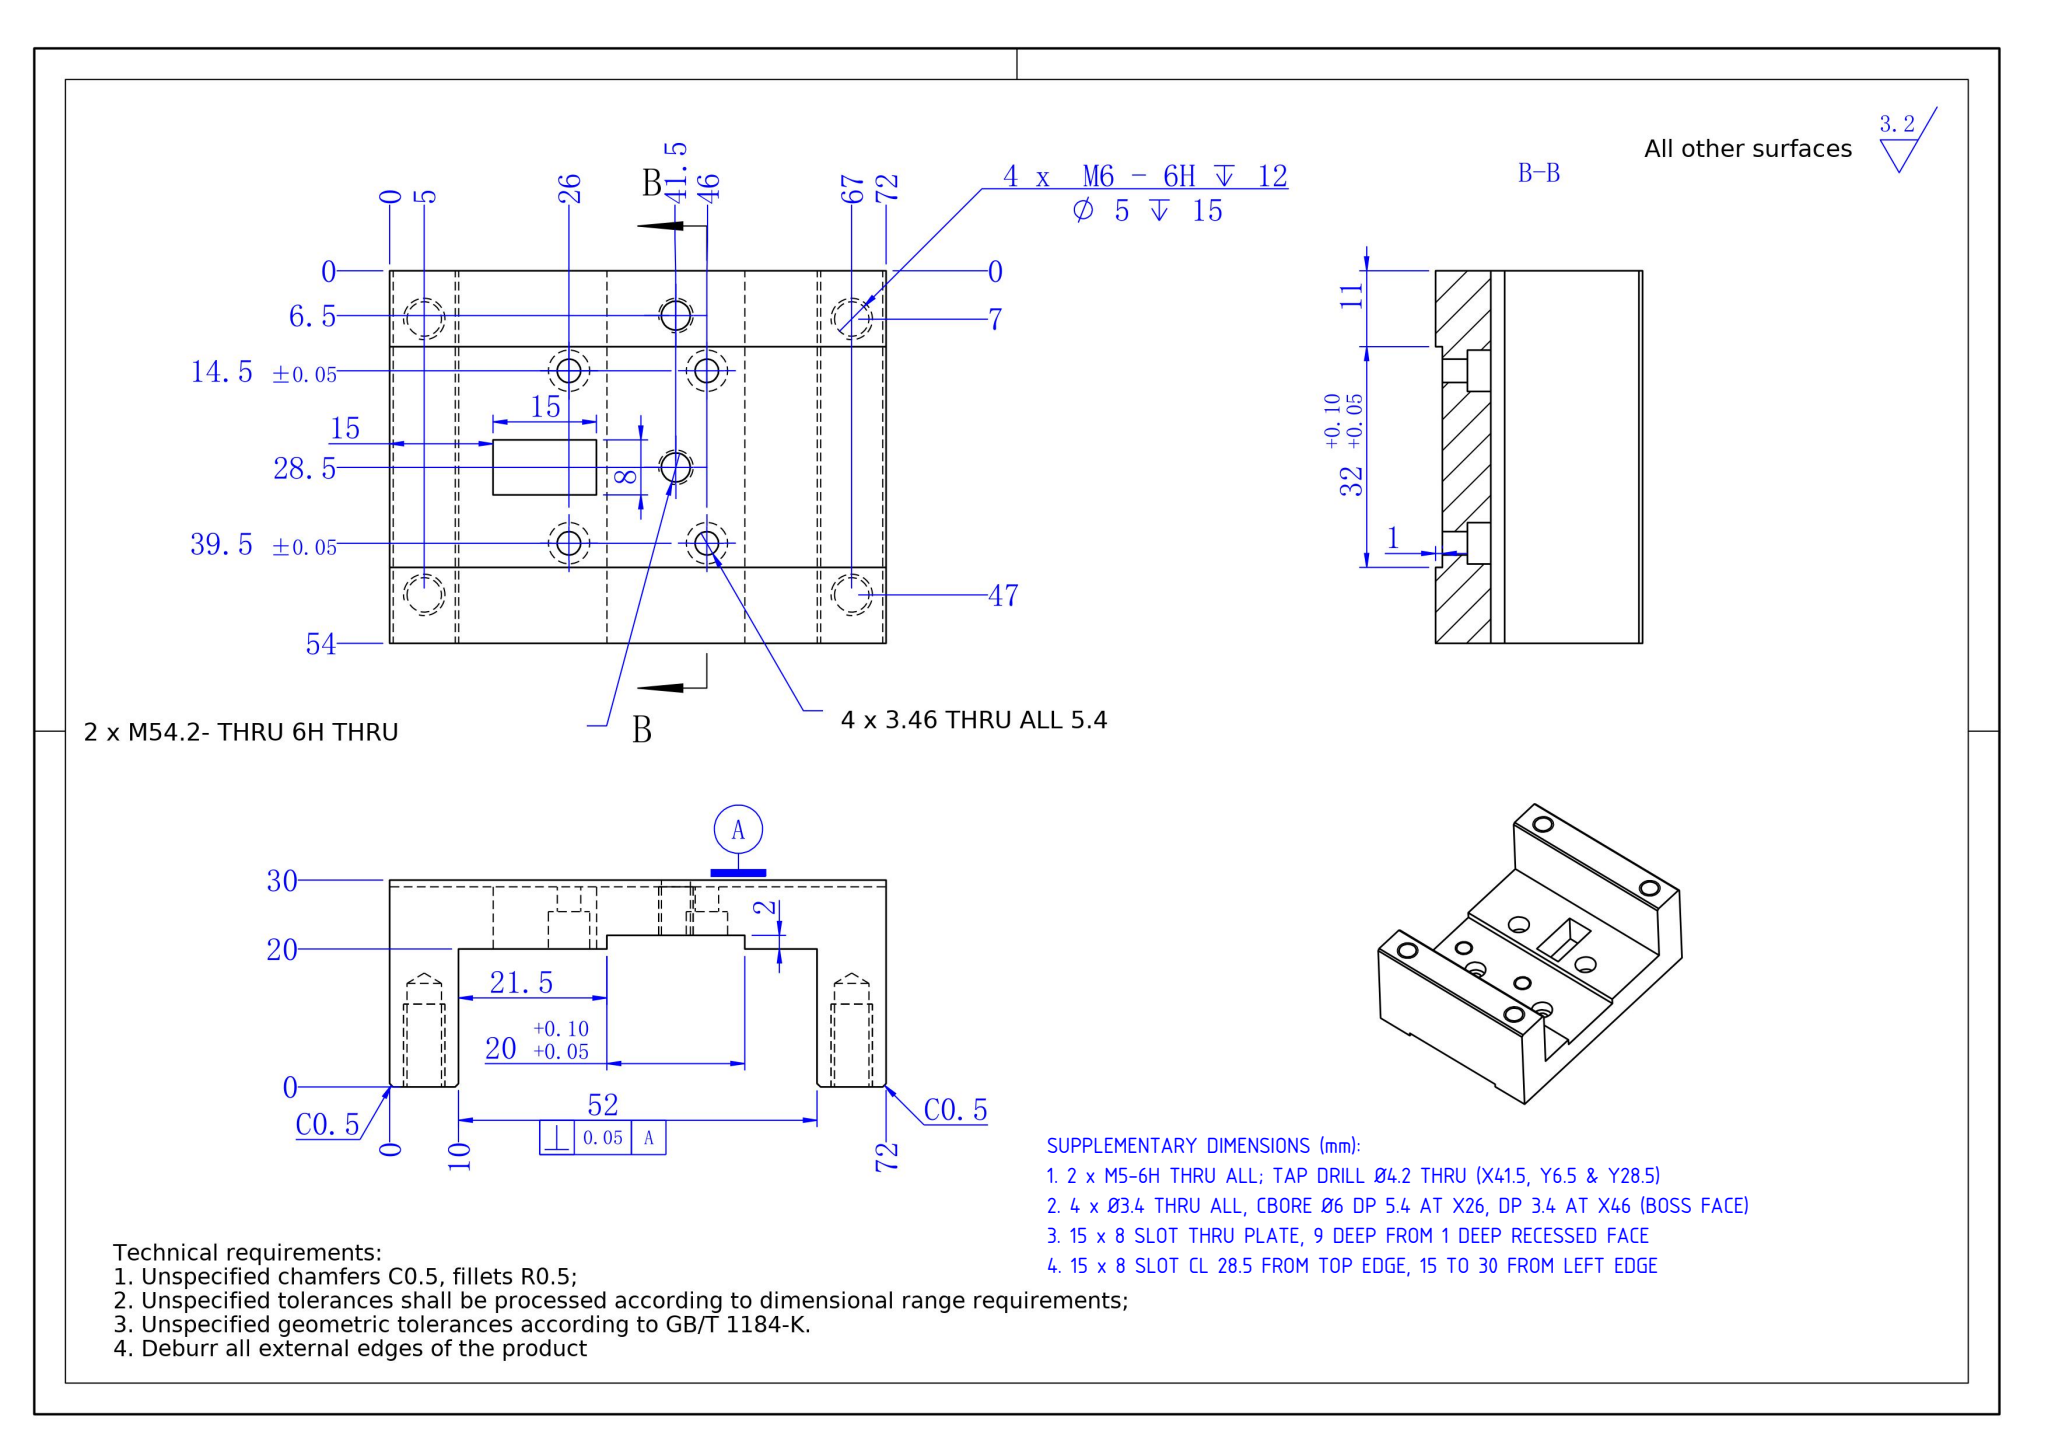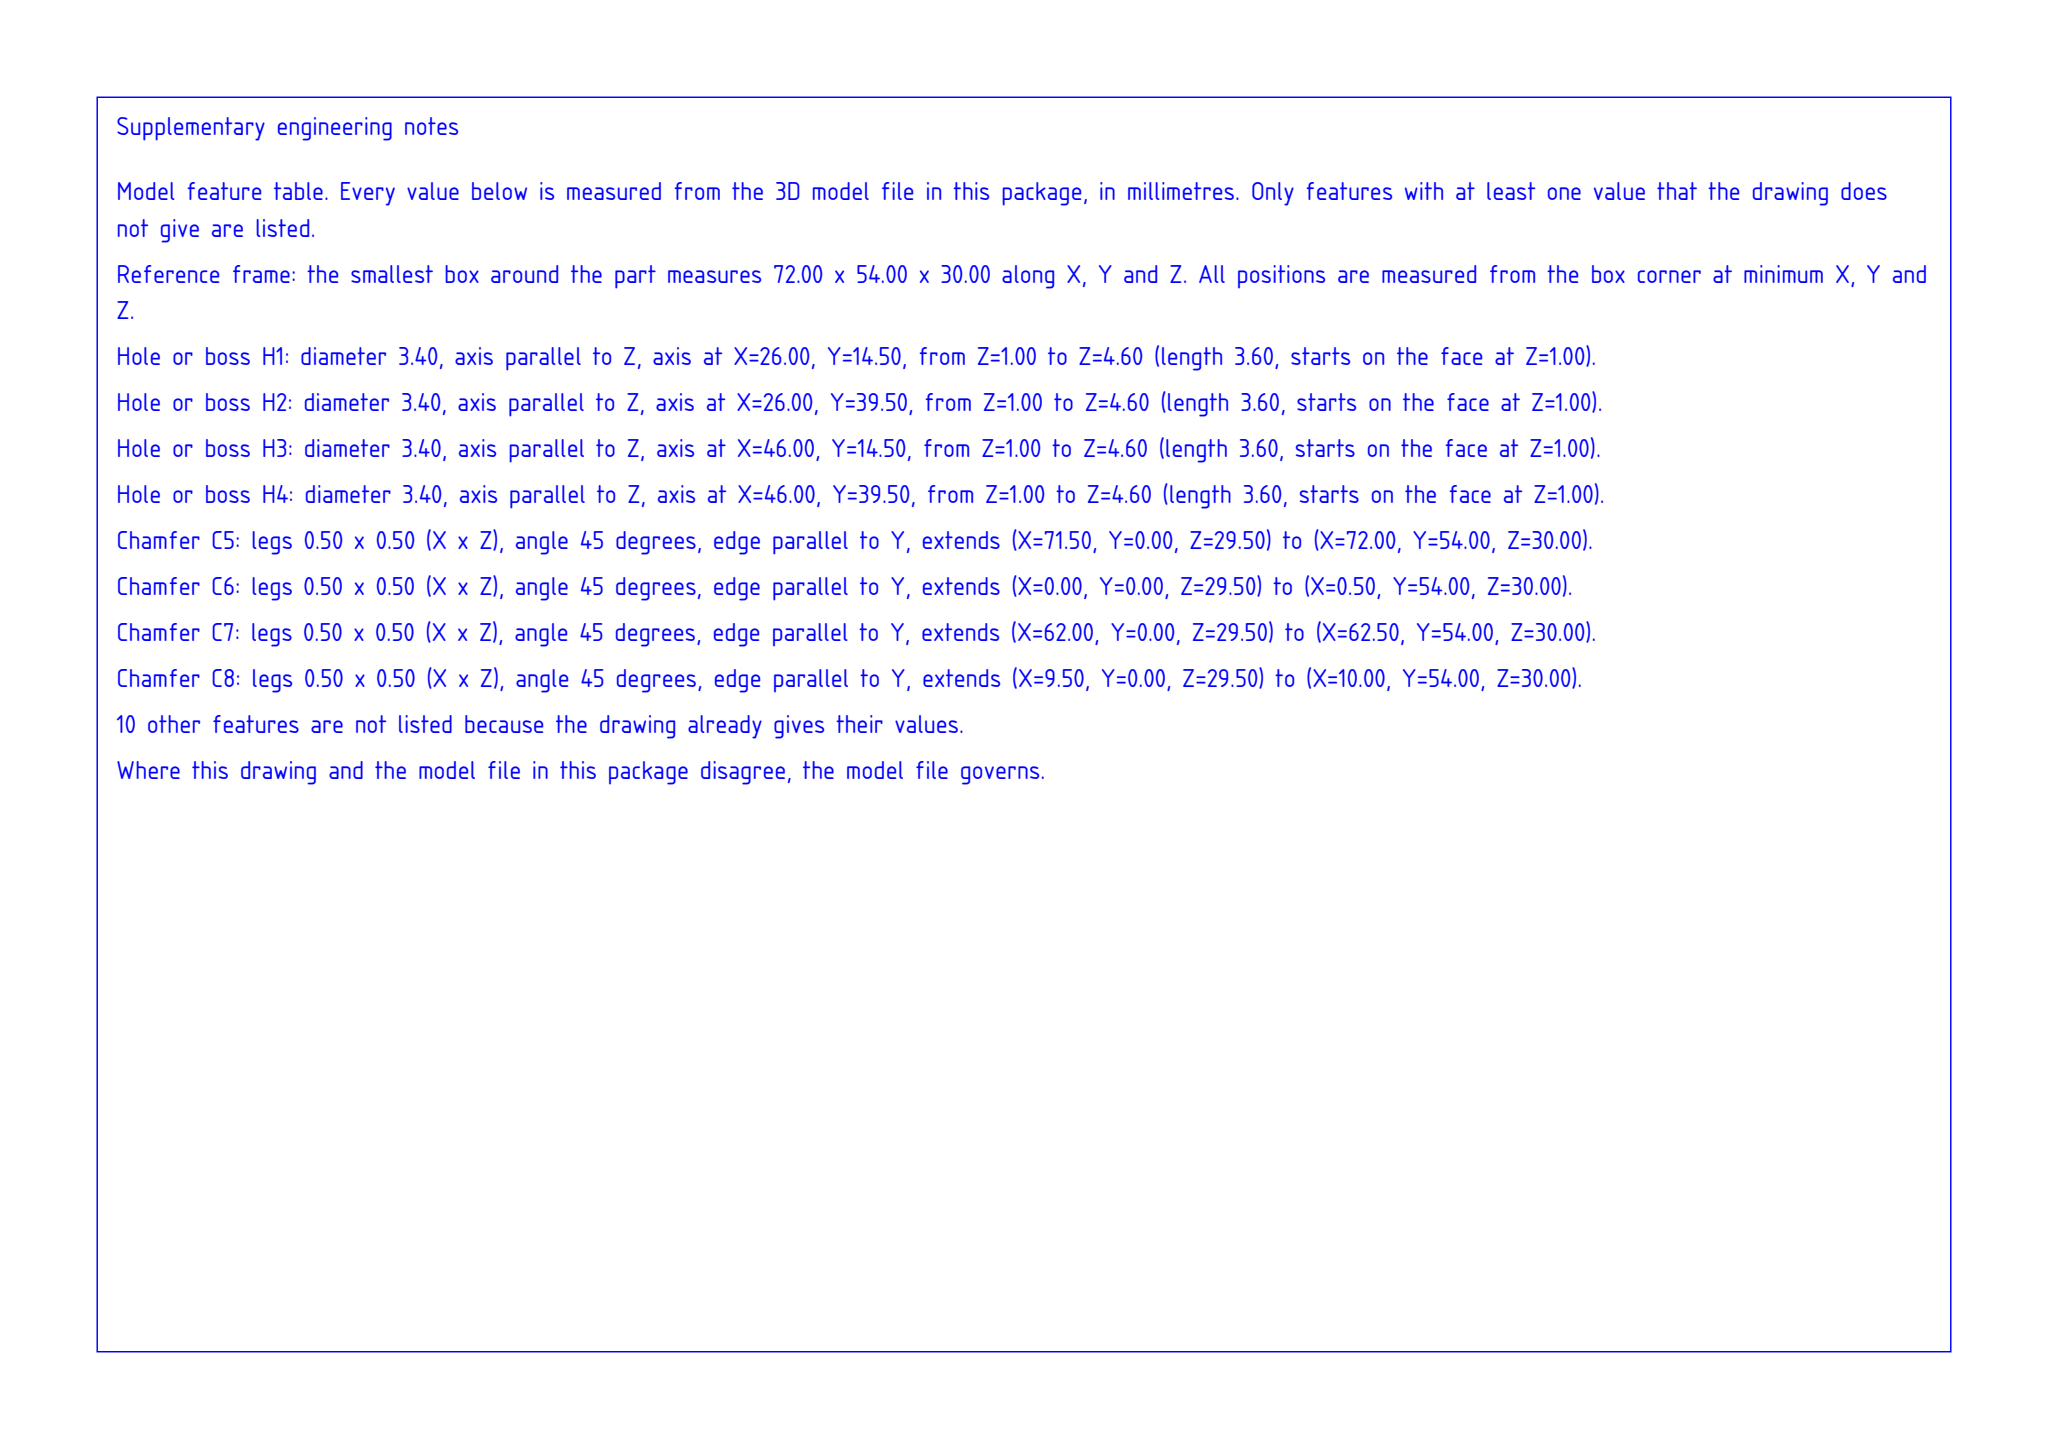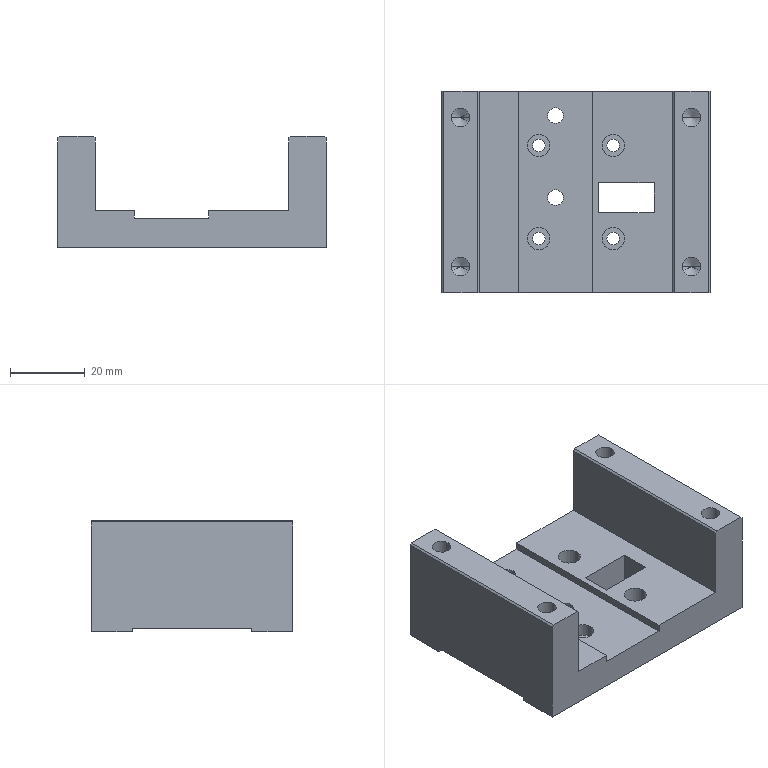Part | SolidWorks | mm | 1 solid | 66 faces | box 72 x 54 x 30 mm | volume 52855 mm3 | plane 30 | cylinder 28 | cone 8 | commonest cylinder face diameters 6 x8 3.4 x8 5 x8 4.2 x4
build123d program:
from build123d import *

# Parameters (mm, degrees)
SKETCH1_W                                          = 72
SKETCH1_H                                          = 54
BOSS_EXTRUDE1_DEPTH                                = 30
M6_TAPPED_HOLE1_D                                  = 5
M6_TAPPED_HOLE1_DEPTH                              = 15
M6_TAPPED_HOLE1_TIP                                = 1.502
SKETCH6_W                                          = 52
SKETCH6_H                                          = 96.611
CUT_EXTRUDE1_DEPTH                                 = 20
SKETCH9_W                                          = 72
SKETCH9_H                                          = 32
CUT_EXTRUDE2_DEPTH                                 = 1
CHAMFER2_SIZE                                      = 0.5
HOLE_SIZE_ACCORDING_TO_TYPE_OF_HEX_SOC_D           = 3.4
HOLE_SIZE_ACCORDING_TO_TYPE_OF_HEX_SOC_CBORE_D     = 6
HOLE_SIZE_ACCORDING_TO_TYPE_OF_HEX_SOC_CBORE_DEPTH = 5.4
SKETCH16_W                                         = 20
SKETCH16_H                                         = 2
CUT_EXTRUDE3_DEPTH                                 = 95.868
M5_TAPPED_HOLE2_D                                  = 4.2
SKETCH19_W                                         = 15
SKETCH19_H                                         = 8
CUT_EXTRUDE4_DEPTH                                 = 52


with BuildPart() as part:
    # Sketch1 → Boss-Extrude1 (new body)
    with BuildSketch(Plane.XY):
        with Locations((36, 27)):
            Rectangle(SKETCH1_W, SKETCH1_H)
    extrude(amount=BOSS_EXTRUDE1_DEPTH)

    # M6 Tapped Hole1
    with Locations(Plane.XY.offset(30)):
        with Locations((5, 47), (67, 47), (67, 7), (5, 7)):
            Hole(M6_TAPPED_HOLE1_D / 2, depth=M6_TAPPED_HOLE1_DEPTH)
            with Locations((0, 0, -(M6_TAPPED_HOLE1_DEPTH + M6_TAPPED_HOLE1_TIP / 2))):  # 118° drill point
                Cone(0, M6_TAPPED_HOLE1_D / 2, M6_TAPPED_HOLE1_TIP, mode=Mode.SUBTRACT)

    # Sketch6 → Cut-Extrude1 (cut)
    with BuildSketch(Plane.XY.offset(30)):
        with Locations((36, 34.886)):
            Rectangle(SKETCH6_W, SKETCH6_H)
    extrude(amount=-CUT_EXTRUDE1_DEPTH, mode=Mode.SUBTRACT)

    # Sketch9 → Cut-Extrude2 (cut)
    with BuildSketch(Plane(origin=(0, 0, 0), x_dir=(-1, 0, 0), z_dir=(0, 0, -1))):
        with Locations((-36, 27)):
            Rectangle(SKETCH9_W, SKETCH9_H)
    extrude(amount=-CUT_EXTRUDE2_DEPTH, mode=Mode.SUBTRACT)

    # Chamfer2
    chamfer2_edges = [part.edges().sort_by_distance(p)[0] for p in [
        (72, 27, 30),
        (10, 27, 30),
        (62, 27, 30),
        (0, 27, 30),
    ]]
    chamfer(chamfer2_edges, length=CHAMFER2_SIZE)

    # Hole Size _according to_ Type of Hex Soc (through all)
    with Locations(Plane.XY.offset(10)):
        with Locations((46, 14.5), (26, 14.5), (46, 39.5), (26, 39.5)):
            CounterBoreHole(HOLE_SIZE_ACCORDING_TO_TYPE_OF_HEX_SOC_D / 2, HOLE_SIZE_ACCORDING_TO_TYPE_OF_HEX_SOC_CBORE_D / 2, HOLE_SIZE_ACCORDING_TO_TYPE_OF_HEX_SOC_CBORE_DEPTH)

    # Sketch16 → Cut-Extrude3 (cut, through all)
    with BuildSketch(Plane(origin=(0, 54, 0), x_dir=(1, 0, 0), z_dir=(0, 1, 0))):
        with Locations((30.5, -9)):
            Rectangle(SKETCH16_W, SKETCH16_H)
    extrude(amount=-CUT_EXTRUDE3_DEPTH, mode=Mode.SUBTRACT)

    # M5 Tapped Hole2 (through all)
    with Locations(Plane.XY.offset(8)):
        with Locations((30.5, 47.5), (30.5, 25.5)):
            Hole(M5_TAPPED_HOLE2_D / 2)

    # Sketch19 → Cut-Extrude4 (cut)
    with BuildSketch(Plane.XY.offset(10)):
        with Locations((49.5, 25.5)):
            Rectangle(SKETCH19_W, SKETCH19_H)
    extrude(amount=-CUT_EXTRUDE4_DEPTH, mode=Mode.SUBTRACT)


solid = part.part